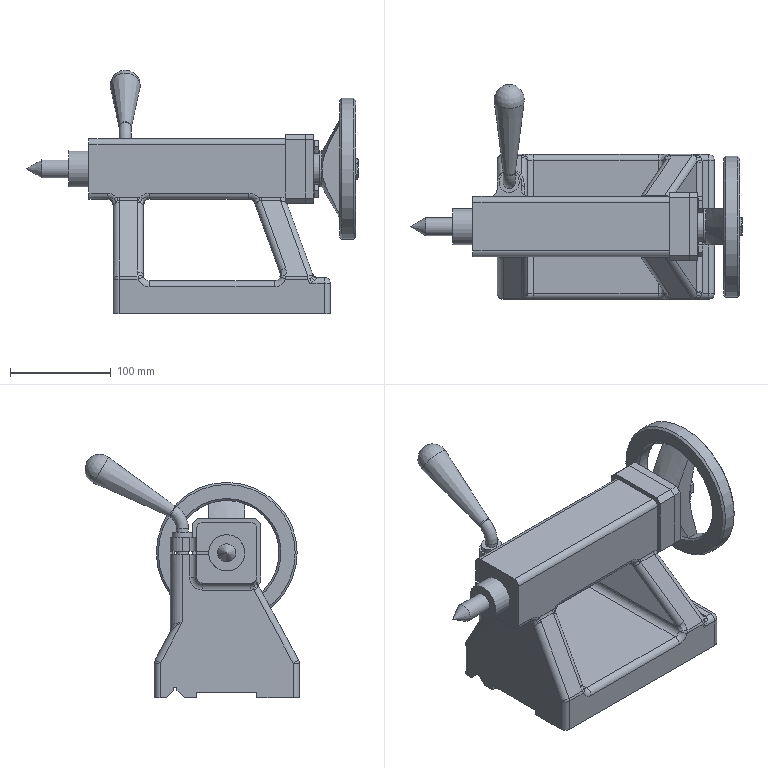Assembly | NX | mm | 15 component files | 15 solids | 386 faces | box 329.89 x 213.27 x 242 mm | volume 2546981 mm3 | plane 164 | cylinder 94 | cone 59 | spline 39 | torus 18 | sphere 12 | commonest cylinder face diameters 12 x36 14 x10 7.76 x8 36 x5 9 x4 20 x4 24 x4 4 x4
Bill of materials:
unnamed part 1 | 1 |  | Bent handle: a short straight cylindrical stem with a thin raised collar, which curves into a long tapered arm. The arm widens toward a rounded, bulb-shaped free end.
unnamed part 2 | 1 |  | Long stepped round shaft: a long main body, a narrow raised collar, then several smaller-diameter steps down to one end. One of the reduced steps has a closed-end slot along its length.
unnamed part 3 | 1 |  | Solid bar with a rounded-end (stadium-shaped) outline: flat top and bottom faces, straight parallel sides and fully rounded ends.
unnamed part 4 | 1 |  | Spoked wheel: a round rim with a rectangular cross-section, a single bar spoke running straight across the full diameter, and a central hub with a round bore and a small keyway notch. The spoke slopes toward the hub, which sits offset from the rim's plane.
unnamed part 5 | 1 |  | Bracket or housing that looks cast: a rectangular box-shaped beam sits on top of a supporting frame with an open window, joined to a rectangular base. One end of the beam is a square flange with a large central bore and four small holes near the corners. The base widens toward the bottom (trapezoid-shaped in end view), has a diagonal rib, and has a small rounded lug with a hole.
GB-T848-2002,M12 | 1 |  | Flat annular ring (plain washer-like shape): a thin disc with a concentric through-hole, flat parallel faces, and plain cylindrical outer and inner edges.
unnamed part 6 | 1 |  | Round pin or rod with a cone-shaped point at one end and a flat face at the other. The shank looks slightly tapered, becoming a little thinner toward the flat end after a short straight section.
unnamed part 7 | 1 |  | Straight round tube or sleeve with a concentric through-bore and a very small notch at one end.
GB-T6170_F-2000,M12x1.75 | 1 |  | Hex nut-shaped body: a six-sided prism with a plain round through-bore and chamfered corners on both faces, giving curved edges on the flat sides.
GB-T5782-2000,M8x16 | 4 |  | Hexagon Head Bolt, GB-T 5782-2000,M8x16
unnamed part 8 | 1 |  | T-shaped part: a solid cylinder with a rectangular block fixed across one end, the block running perpendicular to the cylinder's axis and wider than its diameter in one direction.
unnamed part 9 | 1 |  | Flanged bushing: a square plate with chamfered corners, four through-holes near the corners and a central through-bore. Cylindrical bosses of two different diameters stick out from the two faces.
Mates:
1. fix | frame 1 component
2. touch align | live_center 1 face | slide_sleeve 1 face
3. touch align | live_center 1 face | slide_sleeve 1 face
4. distance | slide_sleeve 1 face | frame 1 face
5. touch align | slide_sleeve 1 face | frame 1 face
6. concentric | lead_screw 1 edge | end_cap 1 edge
7. concentric | end_cap 1 edge | frame 1 edge
8. concentric | flat_key 1 edge | lead_screw 1 edge
9. concentric | lock_handle 1 edge | frame 1 edge
10. touch align | detent_pin 1 face | frame 1 face
11. touch align | detent_pin 1 face | slide_sleeve 1 face
12. concentric | handle 1 edge | end_cap 1 edge
13. concentric | GB-T848-2002_M12 1 edge | handle 1 edge
14. concentric | GB-T6170_F-2000_M12x1_75 1 edge | GB-T848-2002_M12 1 edge